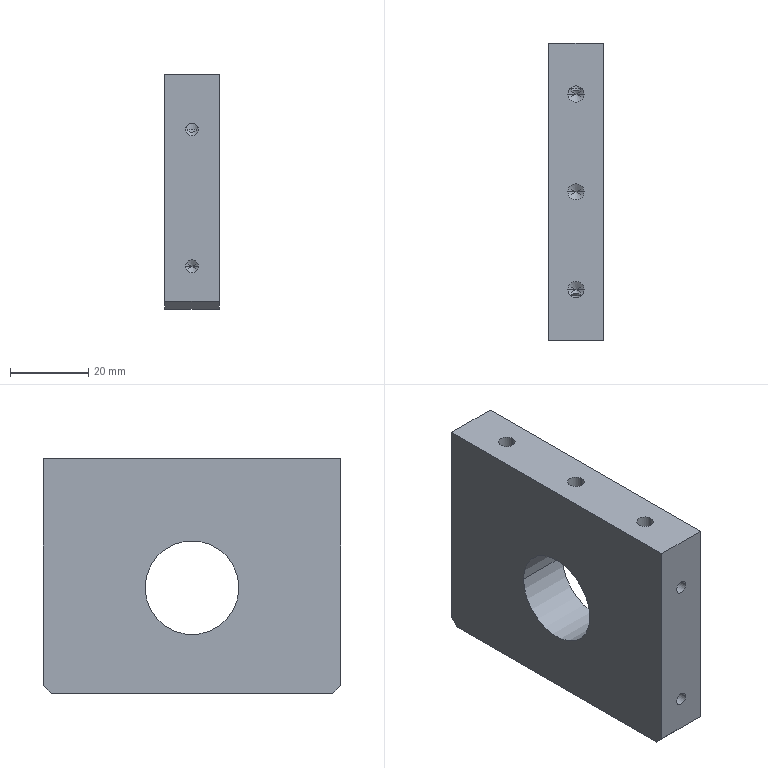Component | SolidWorks | VerticalRearSeat-2-1 | 1 solid | 40 faces | box 14 x 76 x 60 mm | volume 56454 mm3 | cylinder 16 | cone 16 | plane 8 | commonest cylinder face diameters 3.3 x8 4.2 x6 24 x2
build123d program:
from build123d import *

# Parameters (mm, degrees)
SKETCH1_W             = 76
SKETCH1_H             = 60
SKETCH1_R             = 12
BOSS_EXTRUDE1_DEPTH   = 14
CHAMFER1_SIZE         = 2
M5_TAPPED_HOLE1_D     = 4.2
M5_TAPPED_HOLE1_DEPTH = 14
M5_TAPPED_HOLE1_TIP   = 1.262
M4_TAPPED_HOLE1_D     = 3.3
M4_TAPPED_HOLE1_DEPTH = 11.5
M4_TAPPED_HOLE1_TIP   = 0.9914
M4_TAPPED_HOLE2_D     = 3.3
M4_TAPPED_HOLE2_DEPTH = 11.5
M4_TAPPED_HOLE2_TIP   = 0.9914


with BuildPart() as part:
    # Sketch1 → Boss-Extrude1 (new body)
    with BuildSketch(Plane.XY):
        with Locations((38, 30)):
            Rectangle(SKETCH1_W, SKETCH1_H)
        with Locations((38, 33)):
            Circle(SKETCH1_R, mode=Mode.SUBTRACT)
    extrude(amount=BOSS_EXTRUDE1_DEPTH)

    # Chamfer1
    chamfer1_edges = [part.edges().sort_by_distance(p)[0] for p in [
        (0, 60, 7),
        (76, 60, 7),
    ]]
    chamfer(chamfer1_edges, length=CHAMFER1_SIZE)

    # M5 Tapped Hole1
    with Locations(Plane(origin=(0, 0, 0), x_dir=(-1, 0, 0), z_dir=(0, -1, 0))):
        with Locations((-63, -7), (-38, -7), (-13, -7)):
            Hole(M5_TAPPED_HOLE1_D / 2, depth=M5_TAPPED_HOLE1_DEPTH)
            with Locations((0, 0, -(M5_TAPPED_HOLE1_DEPTH + M5_TAPPED_HOLE1_TIP / 2))):  # 118° drill point
                Cone(0, M5_TAPPED_HOLE1_D / 2, M5_TAPPED_HOLE1_TIP, mode=Mode.SUBTRACT)

    # M4 Tapped Hole1
    with Locations(Plane(origin=(76, 0, 0), x_dir=(0, 0, -1), z_dir=(1, 0, 0))):
        with Locations((-7, 49), (-7, 14)):
            Hole(M4_TAPPED_HOLE1_D / 2, depth=M4_TAPPED_HOLE1_DEPTH)
            with Locations((0, 0, -(M4_TAPPED_HOLE1_DEPTH + M4_TAPPED_HOLE1_TIP / 2))):  # 118° drill point
                Cone(0, M4_TAPPED_HOLE1_D / 2, M4_TAPPED_HOLE1_TIP, mode=Mode.SUBTRACT)

    # M4 Tapped Hole2
    with Locations(Plane.ZY):
        with Locations((7, 49), (7, 14)):
            Hole(M4_TAPPED_HOLE2_D / 2, depth=M4_TAPPED_HOLE2_DEPTH)
            with Locations((0, 0, -(M4_TAPPED_HOLE2_DEPTH + M4_TAPPED_HOLE2_TIP / 2))):  # 118° drill point
                Cone(0, M4_TAPPED_HOLE2_D / 2, M4_TAPPED_HOLE2_TIP, mode=Mode.SUBTRACT)


solid = part.part

# Placed as in the assembly
solid = solid.moved(Location((-195.522, 57.945, 36.551), (-90, 90, 0)))